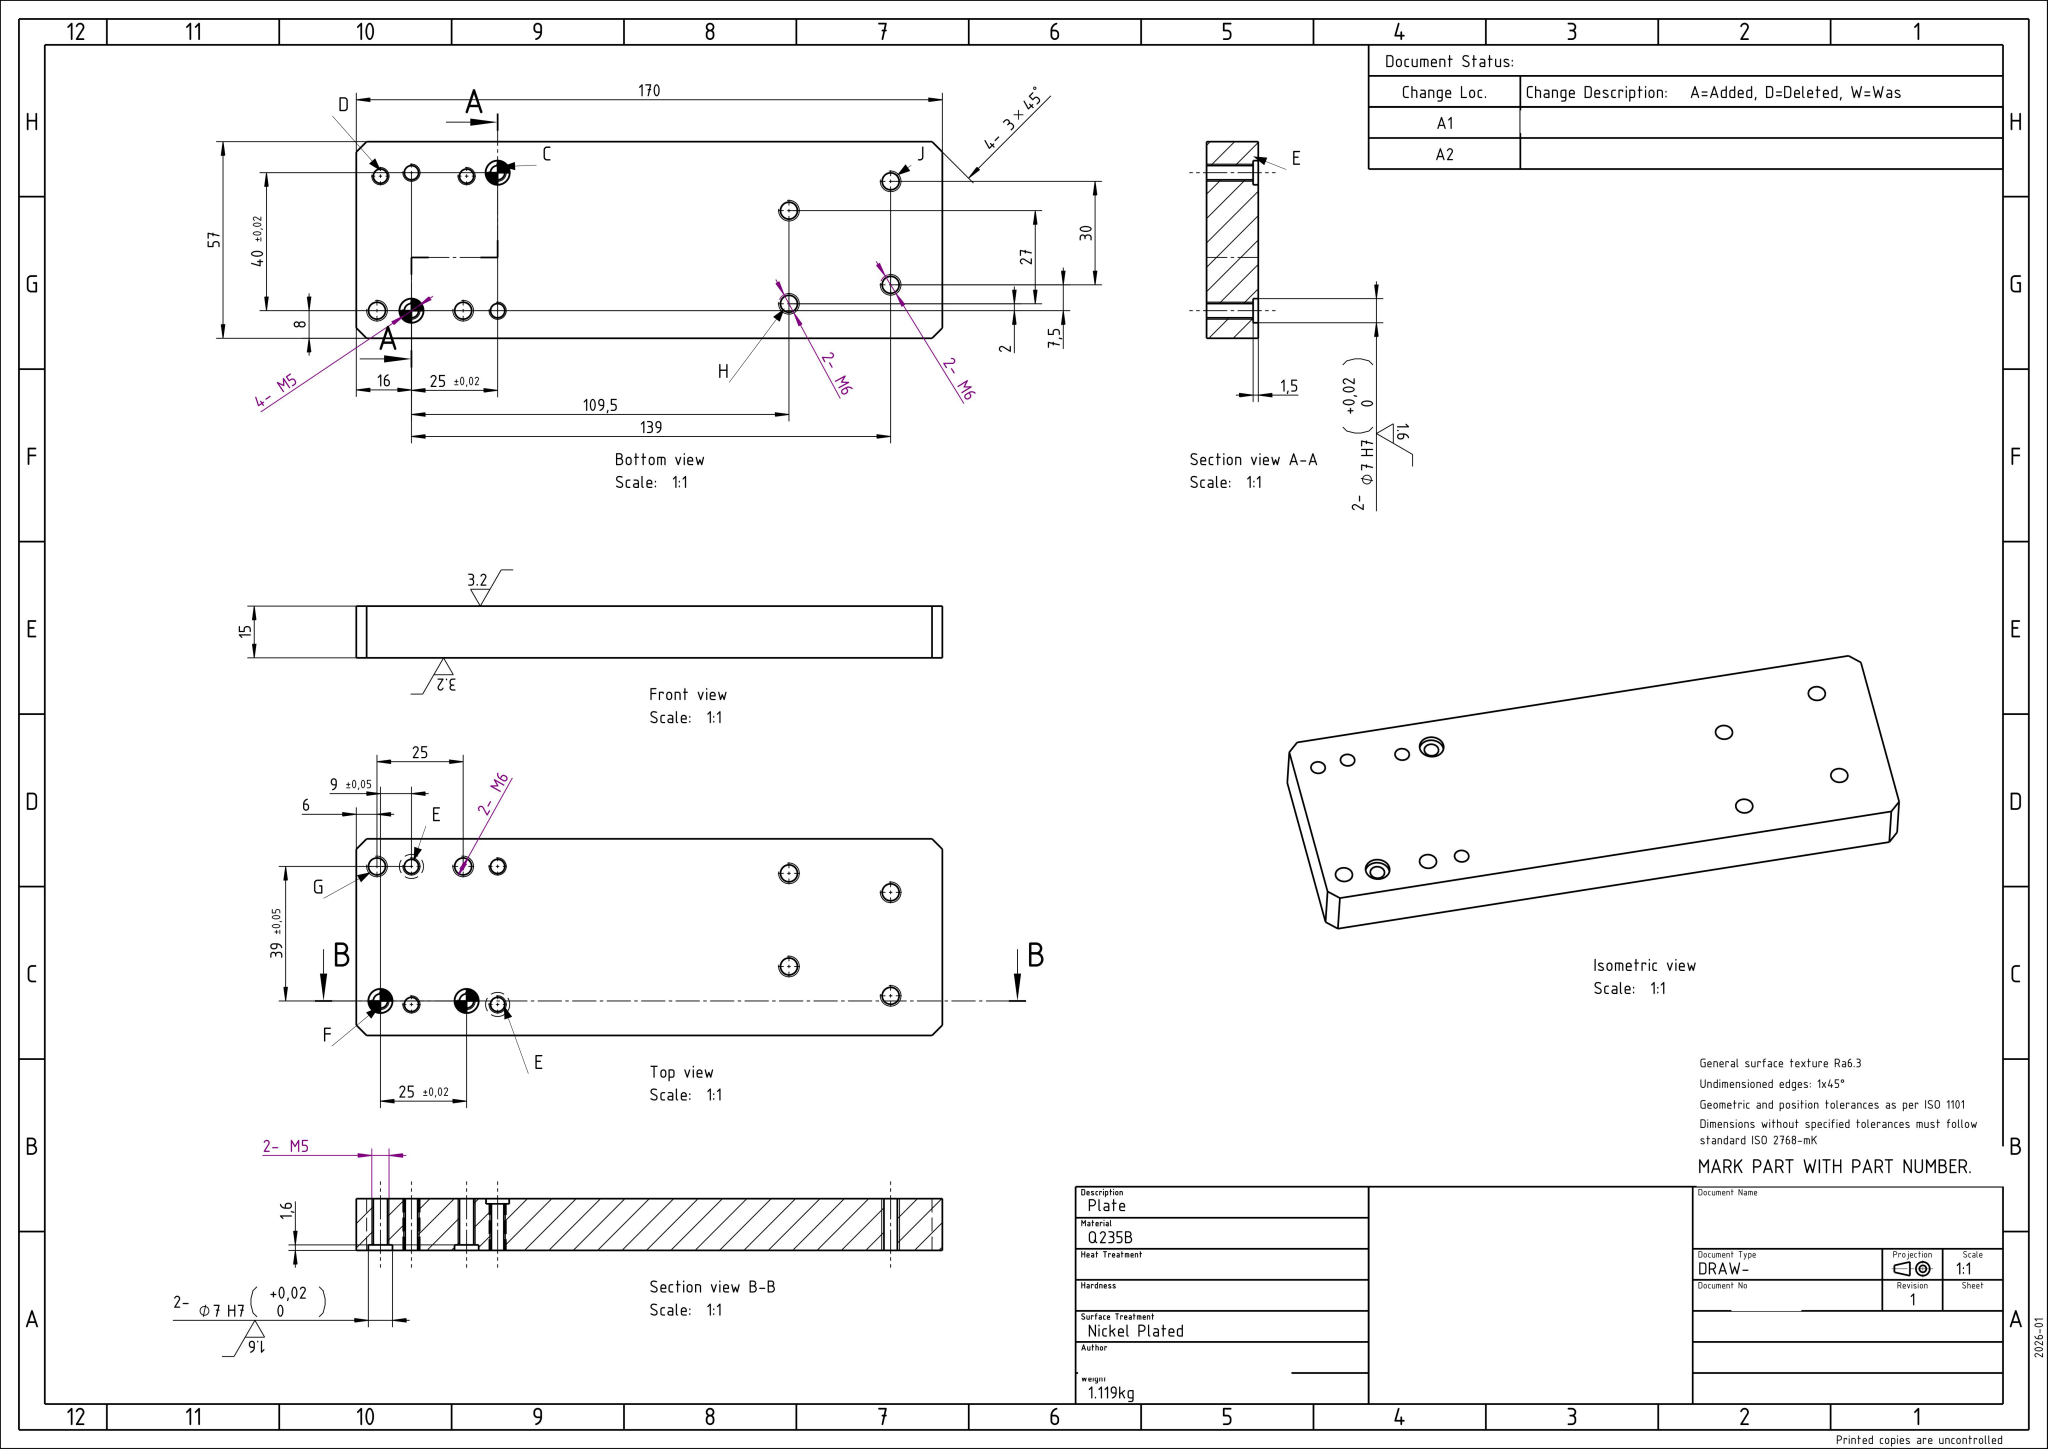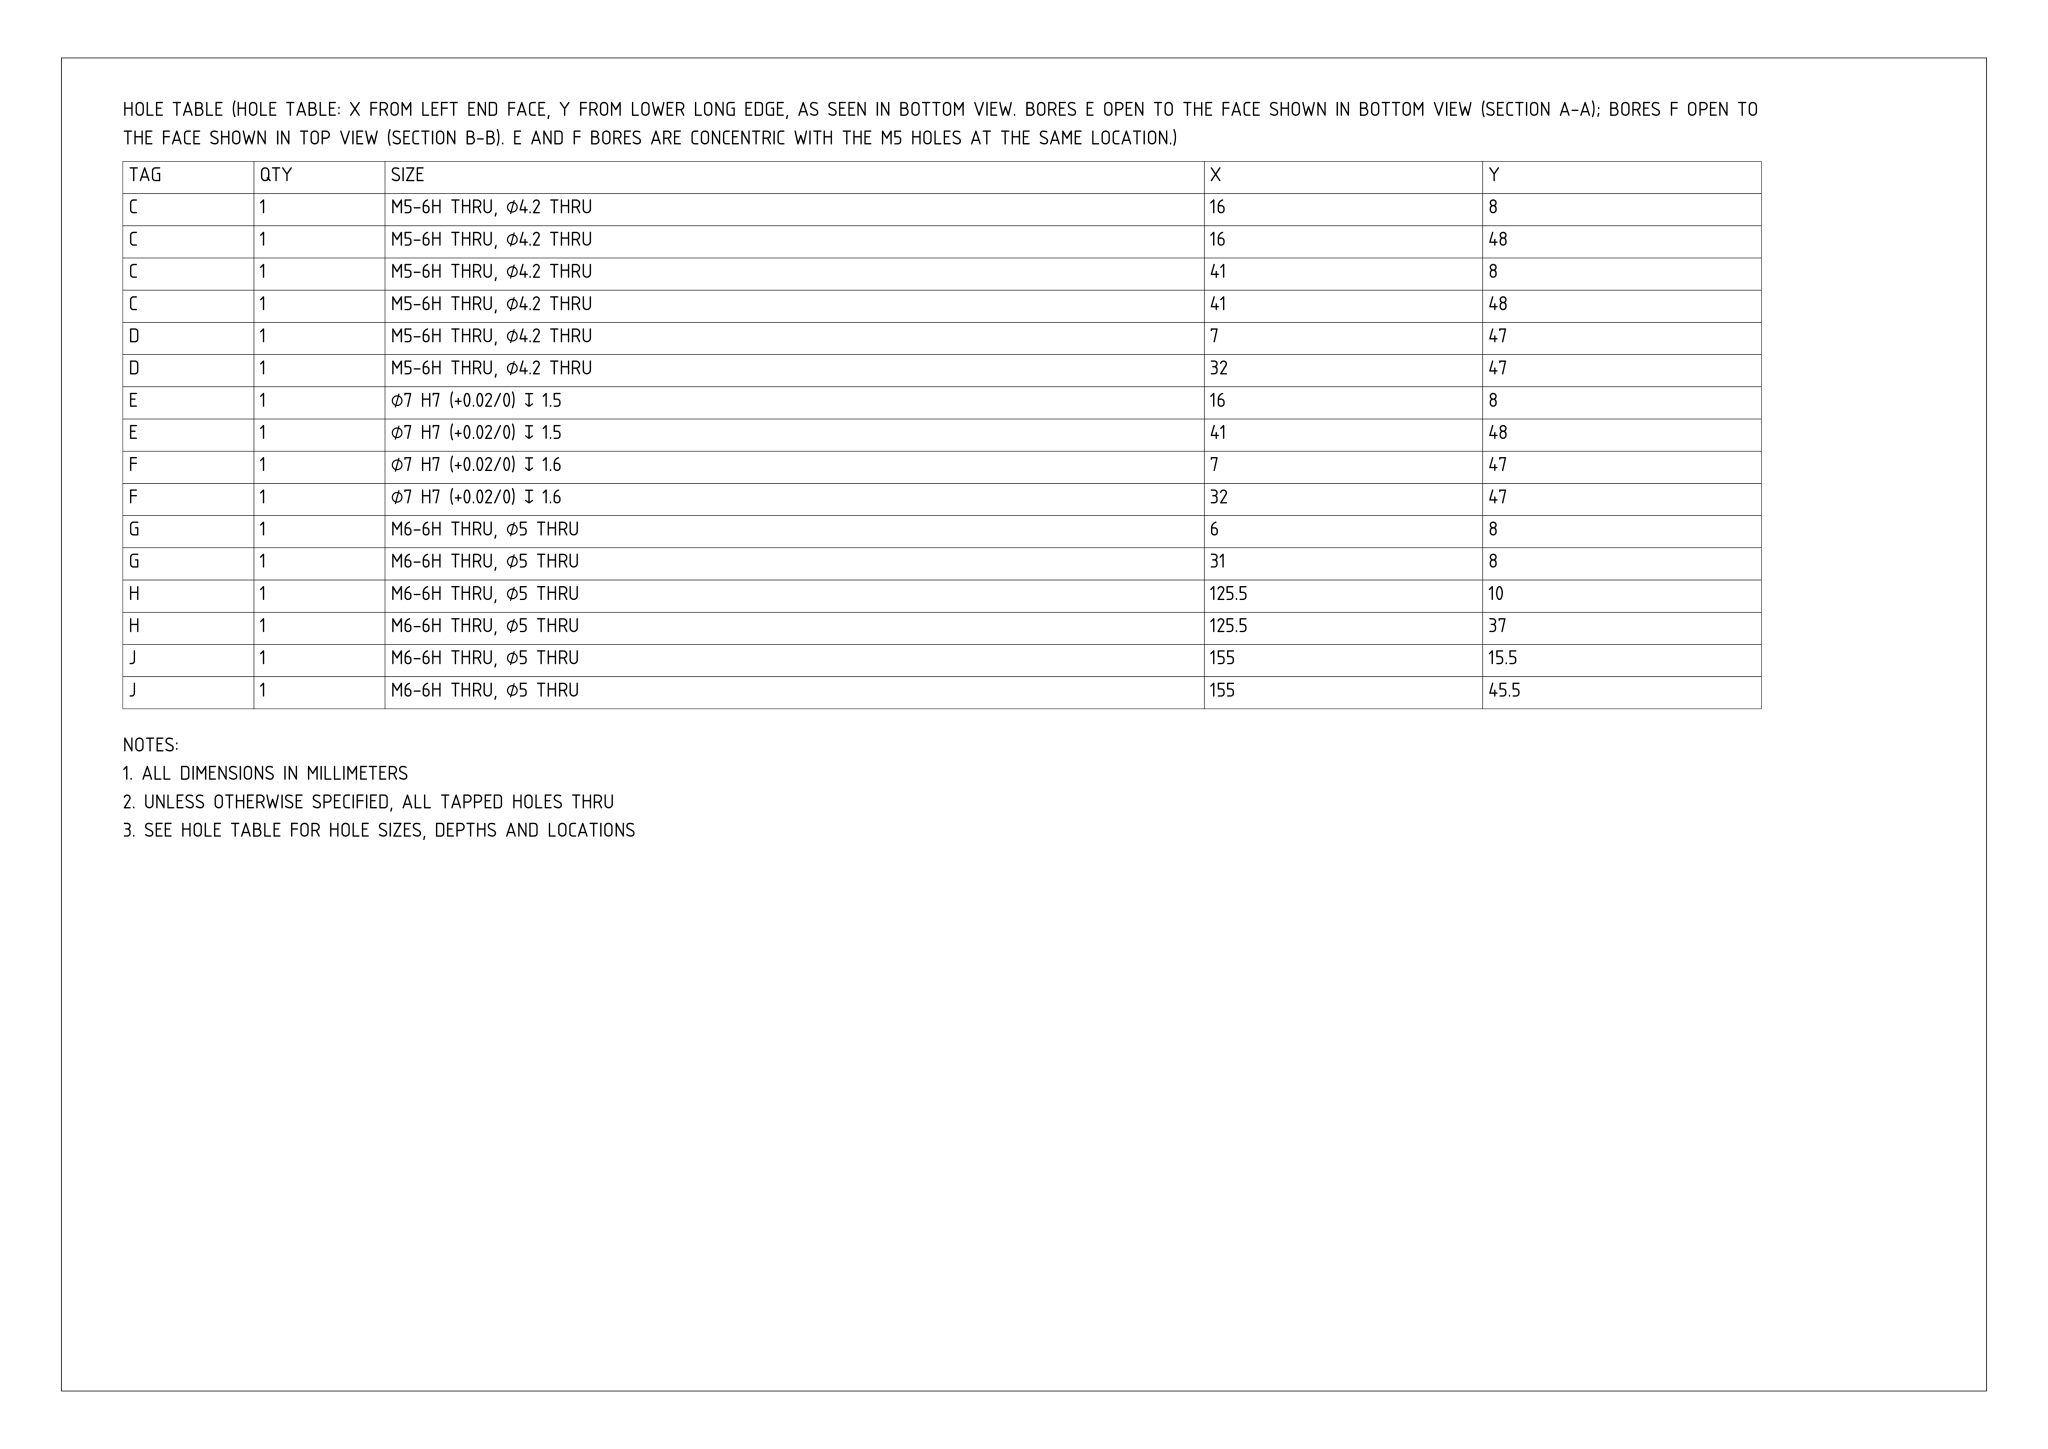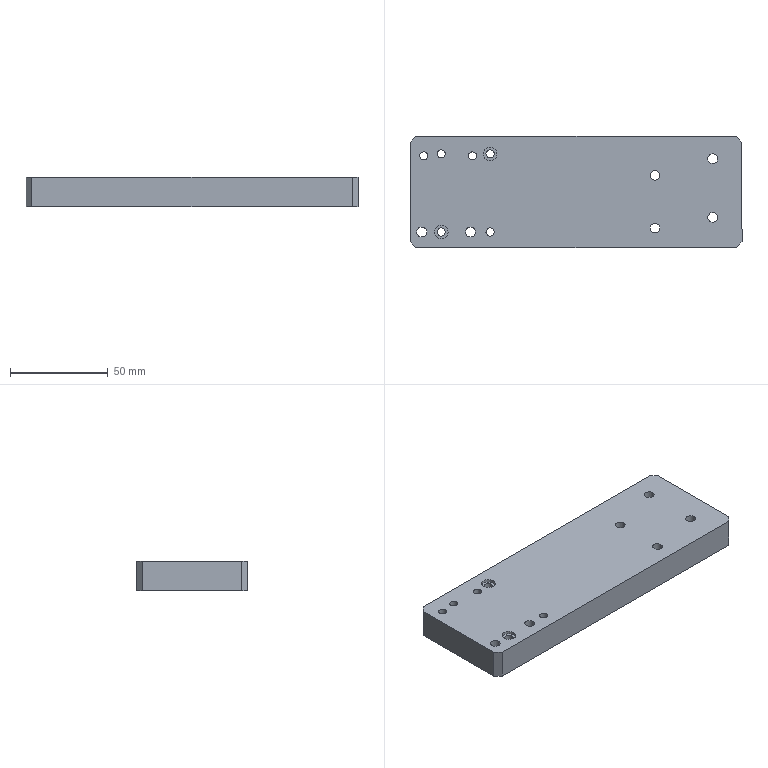Part | NX | mm | 1 solid | 30 faces | box 170 x 57 x 15 mm | volume 141913 mm3 | cylinder 16 | plane 14 | commonest cylinder face diameters 4.2 x6 5 x6 7 x4
STEP:
#1=CARTESIAN_POINT('',(0.,0.,0.));
#2=DIRECTION('',(0.,0.,1.));
#3=DIRECTION('',(1.,0.,0.));
#4=AXIS2_PLACEMENT_3D('',#1,#2,#3);
#5=(LENGTH_UNIT()NAMED_UNIT(*)SI_UNIT(.MILLI.,.METRE.));
#6=UNCERTAINTY_MEASURE_WITH_UNIT(LENGTH_MEASURE(0.00002),#5,'','');
#7=(NAMED_UNIT(*)PLANE_ANGLE_UNIT()SI_UNIT($,.RADIAN.));
#8=PLANE_ANGLE_MEASURE_WITH_UNIT(PLANE_ANGLE_MEASURE(0.01745),#7);
#9=DIMENSIONAL_EXPONENTS(0.,0.,0.,0.,0.,0.,0.);
#10=(CONVERSION_BASED_UNIT('',#8)NAMED_UNIT(#9)PLANE_ANGLE_UNIT());
#11=(NAMED_UNIT(*)SI_UNIT($,.STERADIAN.)SOLID_ANGLE_UNIT());
#12=(GEOMETRIC_REPRESENTATION_CONTEXT(3)GLOBAL_UNCERTAINTY_ASSIGNED_CONTEXT((#6))GLOBAL_UNIT_ASSIGNED_CONTEXT((#5,#10,#11))REPRESENTATION_CONTEXT('',''));
#13=SHAPE_REPRESENTATION('',(#4),#12);
#14=CARTESIAN_POINT('',(-85.,25.5,15.));
#15=VERTEX_POINT('',#14);
#16=CARTESIAN_POINT('',(-85.,-25.5,15.));
#17=VERTEX_POINT('',#16);
#18=CARTESIAN_POINT('',(-85.,28.5,15.));
#19=DIRECTION('',(0.,-1.,0.));
#20=VECTOR('',#19,1.);
#21=LINE('',#18,#20);
#22=EDGE_CURVE('',#15,#17,#21,.T.);
#23=ORIENTED_EDGE('',*,*,#22,.F.);
#24=CARTESIAN_POINT('',(-85.,25.5,0.));
#25=VERTEX_POINT('',#24);
#26=CARTESIAN_POINT('',(-85.,25.5,15.));
#27=DIRECTION('',(0.,0.,-1.));
#28=VECTOR('',#27,1.);
#29=LINE('',#26,#28);
#30=EDGE_CURVE('',#15,#25,#29,.T.);
#31=ORIENTED_EDGE('',*,*,#30,.T.);
#32=CARTESIAN_POINT('',(-85.,-25.5,0.));
#33=VERTEX_POINT('',#32);
#34=CARTESIAN_POINT('',(-85.,28.5,0.));
#35=DIRECTION('',(0.,-1.,0.));
#36=VECTOR('',#35,1.);
#37=LINE('',#34,#36);
#38=EDGE_CURVE('',#25,#33,#37,.T.);
#39=ORIENTED_EDGE('',*,*,#38,.T.);
#40=CARTESIAN_POINT('',(-85.,-25.5,15.));
#41=DIRECTION('',(0.,0.,1.));
#42=VECTOR('',#41,1.);
#43=LINE('',#40,#42);
#44=EDGE_CURVE('',#33,#17,#43,.T.);
#45=ORIENTED_EDGE('',*,*,#44,.T.);
#46=EDGE_LOOP('',(#23,#31,#39,#45));
#47=FACE_OUTER_BOUND('',#46,.T.);
#48=CARTESIAN_POINT('',(-85.,28.5,15.));
#49=DIRECTION('',(1.,0.,0.));
#50=DIRECTION('',(-0.,1.,0.));
#51=AXIS2_PLACEMENT_3D('',#48,#49,#50);
#52=PLANE('',#51);
#53=ADVANCED_FACE('',(#47),#52,.F.);
#54=CARTESIAN_POINT('',(-82.,-28.5,0.));
#55=VERTEX_POINT('',#54);
#56=CARTESIAN_POINT('',(82.,-28.5,0.));
#57=VERTEX_POINT('',#56);
#58=CARTESIAN_POINT('',(-85.,-28.5,0.));
#59=DIRECTION('',(1.,0.,0.));
#60=VECTOR('',#59,1.);
#61=LINE('',#58,#60);
#62=EDGE_CURVE('',#55,#57,#61,.T.);
#63=ORIENTED_EDGE('',*,*,#62,.T.);
#64=CARTESIAN_POINT('',(82.,-28.5,15.));
#65=VERTEX_POINT('',#64);
#66=CARTESIAN_POINT('',(82.,-28.5,15.));
#67=DIRECTION('',(0.,0.,1.));
#68=VECTOR('',#67,1.);
#69=LINE('',#66,#68);
#70=EDGE_CURVE('',#57,#65,#69,.T.);
#71=ORIENTED_EDGE('',*,*,#70,.T.);
#72=CARTESIAN_POINT('',(-82.,-28.5,15.));
#73=VERTEX_POINT('',#72);
#74=CARTESIAN_POINT('',(-85.,-28.5,15.));
#75=DIRECTION('',(1.,0.,0.));
#76=VECTOR('',#75,1.);
#77=LINE('',#74,#76);
#78=EDGE_CURVE('',#73,#65,#77,.T.);
#79=ORIENTED_EDGE('',*,*,#78,.F.);
#80=CARTESIAN_POINT('',(-82.,-28.5,15.));
#81=DIRECTION('',(0.,0.,-1.));
#82=VECTOR('',#81,1.);
#83=LINE('',#80,#82);
#84=EDGE_CURVE('',#73,#55,#83,.T.);
#85=ORIENTED_EDGE('',*,*,#84,.T.);
#86=EDGE_LOOP('',(#63,#71,#79,#85));
#87=FACE_OUTER_BOUND('',#86,.T.);
#88=CARTESIAN_POINT('',(-85.,-28.5,15.));
#89=DIRECTION('',(0.,1.,0.));
#90=DIRECTION('',(0.,0.,1.));
#91=AXIS2_PLACEMENT_3D('',#88,#89,#90);
#92=PLANE('',#91);
#93=ADVANCED_FACE('',(#87),#92,.F.);
#94=CARTESIAN_POINT('',(85.,-25.5,15.));
#95=VERTEX_POINT('',#94);
#96=CARTESIAN_POINT('',(85.,25.5,15.));
#97=VERTEX_POINT('',#96);
#98=CARTESIAN_POINT('',(85.,-28.5,15.));
#99=DIRECTION('',(-0.,1.,0.));
#100=VECTOR('',#99,1.);
#101=LINE('',#98,#100);
#102=EDGE_CURVE('',#95,#97,#101,.T.);
#103=ORIENTED_EDGE('',*,*,#102,.F.);
#104=CARTESIAN_POINT('',(85.,-25.5,0.));
#105=VERTEX_POINT('',#104);
#106=CARTESIAN_POINT('',(85.,-25.5,15.));
#107=DIRECTION('',(0.,0.,-1.));
#108=VECTOR('',#107,1.);
#109=LINE('',#106,#108);
#110=EDGE_CURVE('',#95,#105,#109,.T.);
#111=ORIENTED_EDGE('',*,*,#110,.T.);
#112=CARTESIAN_POINT('',(85.,25.5,0.));
#113=VERTEX_POINT('',#112);
#114=CARTESIAN_POINT('',(85.,-28.5,0.));
#115=DIRECTION('',(-0.,1.,0.));
#116=VECTOR('',#115,1.);
#117=LINE('',#114,#116);
#118=EDGE_CURVE('',#105,#113,#117,.T.);
#119=ORIENTED_EDGE('',*,*,#118,.T.);
#120=CARTESIAN_POINT('',(85.,25.5,15.));
#121=DIRECTION('',(0.,0.,1.));
#122=VECTOR('',#121,1.);
#123=LINE('',#120,#122);
#124=EDGE_CURVE('',#113,#97,#123,.T.);
#125=ORIENTED_EDGE('',*,*,#124,.T.);
#126=EDGE_LOOP('',(#103,#111,#119,#125));
#127=FACE_OUTER_BOUND('',#126,.T.);
#128=CARTESIAN_POINT('',(85.,-28.5,15.));
#129=DIRECTION('',(-1.,-0.,0.));
#130=DIRECTION('',(0.,-1.,0.));
#131=AXIS2_PLACEMENT_3D('',#128,#129,#130);
#132=PLANE('',#131);
#133=ADVANCED_FACE('',(#127),#132,.F.);
#134=CARTESIAN_POINT('',(82.,28.5,0.));
#135=VERTEX_POINT('',#134);
#136=CARTESIAN_POINT('',(-82.,28.5,0.));
#137=VERTEX_POINT('',#136);
#138=CARTESIAN_POINT('',(85.,28.5,0.));
#139=DIRECTION('',(-1.,0.,0.));
#140=VECTOR('',#139,1.);
#141=LINE('',#138,#140);
#142=EDGE_CURVE('',#135,#137,#141,.T.);
#143=ORIENTED_EDGE('',*,*,#142,.T.);
#144=CARTESIAN_POINT('',(-82.,28.5,15.));
#145=VERTEX_POINT('',#144);
#146=CARTESIAN_POINT('',(-82.,28.5,15.));
#147=DIRECTION('',(0.,0.,1.));
#148=VECTOR('',#147,1.);
#149=LINE('',#146,#148);
#150=EDGE_CURVE('',#137,#145,#149,.T.);
#151=ORIENTED_EDGE('',*,*,#150,.T.);
#152=CARTESIAN_POINT('',(82.,28.5,15.));
#153=VERTEX_POINT('',#152);
#154=CARTESIAN_POINT('',(85.,28.5,15.));
#155=DIRECTION('',(-1.,0.,0.));
#156=VECTOR('',#155,1.);
#157=LINE('',#154,#156);
#158=EDGE_CURVE('',#153,#145,#157,.T.);
#159=ORIENTED_EDGE('',*,*,#158,.F.);
#160=CARTESIAN_POINT('',(82.,28.5,15.));
#161=DIRECTION('',(0.,0.,-1.));
#162=VECTOR('',#161,1.);
#163=LINE('',#160,#162);
#164=EDGE_CURVE('',#153,#135,#163,.T.);
#165=ORIENTED_EDGE('',*,*,#164,.T.);
#166=EDGE_LOOP('',(#143,#151,#159,#165));
#167=FACE_OUTER_BOUND('',#166,.T.);
#168=CARTESIAN_POINT('',(85.,28.5,15.));
#169=DIRECTION('',(0.,-1.,0.));
#170=DIRECTION('',(0.,0.,-1.));
#171=AXIS2_PLACEMENT_3D('',#168,#169,#170);
#172=PLANE('',#171);
#173=ADVANCED_FACE('',(#167),#172,.F.);
#174=CARTESIAN_POINT('',(72.5,17.,15.));
#175=VERTEX_POINT('',#174);
#176=CARTESIAN_POINT('',(70.,17.,15.));
#177=DIRECTION('',(0.,0.,1.));
#178=DIRECTION('',(1.,0.,0.));
#179=AXIS2_PLACEMENT_3D('',#176,#177,#178);
#180=CIRCLE('',#179,2.5);
#181=EDGE_CURVE('',#175,#175,#180,.T.);
#182=ORIENTED_EDGE('',*,*,#181,.F.);
#183=EDGE_LOOP('',(#182));
#184=FACE_BOUND('',#183,.T.);
#185=CARTESIAN_POINT('',(72.5,-13.,15.));
#186=VERTEX_POINT('',#185);
#187=CARTESIAN_POINT('',(70.,-13.,15.));
#188=DIRECTION('',(0.,0.,1.));
#189=DIRECTION('',(1.,0.,0.));
#190=AXIS2_PLACEMENT_3D('',#187,#188,#189);
#191=CIRCLE('',#190,2.5);
#192=EDGE_CURVE('',#186,#186,#191,.T.);
#193=ORIENTED_EDGE('',*,*,#192,.F.);
#194=EDGE_LOOP('',(#193));
#195=FACE_BOUND('',#194,.T.);
#196=CARTESIAN_POINT('',(43.,8.5,15.));
#197=VERTEX_POINT('',#196);
#198=CARTESIAN_POINT('',(40.5,8.5,15.));
#199=DIRECTION('',(0.,0.,1.));
#200=DIRECTION('',(1.,0.,0.));
#201=AXIS2_PLACEMENT_3D('',#198,#199,#200);
#202=CIRCLE('',#201,2.5);
#203=EDGE_CURVE('',#197,#197,#202,.T.);
#204=ORIENTED_EDGE('',*,*,#203,.F.);
#205=EDGE_LOOP('',(#204));
#206=FACE_BOUND('',#205,.T.);
#207=CARTESIAN_POINT('',(43.,-18.5,15.));
#208=VERTEX_POINT('',#207);
#209=CARTESIAN_POINT('',(40.5,-18.5,15.));
#210=DIRECTION('',(0.,0.,1.));
#211=DIRECTION('',(1.,0.,0.));
#212=AXIS2_PLACEMENT_3D('',#209,#210,#211);
#213=CIRCLE('',#212,2.5);
#214=EDGE_CURVE('',#208,#208,#213,.T.);
#215=ORIENTED_EDGE('',*,*,#214,.F.);
#216=EDGE_LOOP('',(#215));
#217=FACE_BOUND('',#216,.T.);
#218=CARTESIAN_POINT('',(-50.9,18.5,15.));
#219=VERTEX_POINT('',#218);
#220=CARTESIAN_POINT('',(-53.,18.5,15.));
#221=DIRECTION('',(0.,0.,1.));
#222=DIRECTION('',(1.,0.,0.));
#223=AXIS2_PLACEMENT_3D('',#220,#221,#222);
#224=CIRCLE('',#223,2.1);
#225=EDGE_CURVE('',#219,#219,#224,.T.);
#226=ORIENTED_EDGE('',*,*,#225,.F.);
#227=EDGE_LOOP('',(#226));
#228=FACE_BOUND('',#227,.T.);
#229=CARTESIAN_POINT('',(-75.9,18.5,15.));
#230=VERTEX_POINT('',#229);
#231=CARTESIAN_POINT('',(-78.,18.5,15.));
#232=DIRECTION('',(0.,0.,1.));
#233=DIRECTION('',(1.,0.,0.));
#234=AXIS2_PLACEMENT_3D('',#231,#232,#233);
#235=CIRCLE('',#234,2.1);
#236=EDGE_CURVE('',#230,#230,#235,.T.);
#237=ORIENTED_EDGE('',*,*,#236,.F.);
#238=EDGE_LOOP('',(#237));
#239=FACE_BOUND('',#238,.T.);
#240=CARTESIAN_POINT('',(-56.5,-20.5,15.));
#241=VERTEX_POINT('',#240);
#242=CARTESIAN_POINT('',(-54.,-20.5,15.));
#243=DIRECTION('',(0.,0.,-1.));
#244=DIRECTION('',(-1.,0.,0.));
#245=AXIS2_PLACEMENT_3D('',#242,#243,#244);
#246=CIRCLE('',#245,2.5);
#247=EDGE_CURVE('',#241,#241,#246,.T.);
#248=ORIENTED_EDGE('',*,*,#247,.T.);
#249=EDGE_LOOP('',(#248));
#250=FACE_BOUND('',#249,.T.);
#251=CARTESIAN_POINT('',(-81.5,-20.5,15.));
#252=VERTEX_POINT('',#251);
#253=CARTESIAN_POINT('',(-79.,-20.5,15.));
#254=DIRECTION('',(0.,0.,-1.));
#255=DIRECTION('',(-1.,0.,0.));
#256=AXIS2_PLACEMENT_3D('',#253,#254,#255);
#257=CIRCLE('',#256,2.5);
#258=EDGE_CURVE('',#252,#252,#257,.T.);
#259=ORIENTED_EDGE('',*,*,#258,.T.);
#260=EDGE_LOOP('',(#259));
#261=FACE_BOUND('',#260,.T.);
#262=CARTESIAN_POINT('',(-46.1,-20.5,15.));
#263=VERTEX_POINT('',#262);
#264=CARTESIAN_POINT('',(-44.,-20.5,15.));
#265=DIRECTION('',(0.,0.,-1.));
#266=DIRECTION('',(-1.,0.,0.));
#267=AXIS2_PLACEMENT_3D('',#264,#265,#266);
#268=CIRCLE('',#267,2.1);
#269=EDGE_CURVE('',#263,#263,#268,.T.);
#270=ORIENTED_EDGE('',*,*,#269,.T.);
#271=EDGE_LOOP('',(#270));
#272=FACE_BOUND('',#271,.T.);
#273=CARTESIAN_POINT('',(-71.1,19.5,15.));
#274=VERTEX_POINT('',#273);
#275=CARTESIAN_POINT('',(-69.,19.5,15.));
#276=DIRECTION('',(0.,0.,-1.));
#277=DIRECTION('',(-1.,0.,0.));
#278=AXIS2_PLACEMENT_3D('',#275,#276,#277);
#279=CIRCLE('',#278,2.1);
#280=EDGE_CURVE('',#274,#274,#279,.T.);
#281=ORIENTED_EDGE('',*,*,#280,.T.);
#282=EDGE_LOOP('',(#281));
#283=FACE_BOUND('',#282,.T.);
#284=CARTESIAN_POINT('',(-47.5,19.5,15.));
#285=VERTEX_POINT('',#284);
#286=CARTESIAN_POINT('',(-44.,19.5,15.));
#287=DIRECTION('',(0.,0.,-1.));
#288=DIRECTION('',(-1.,0.,0.));
#289=AXIS2_PLACEMENT_3D('',#286,#287,#288);
#290=CIRCLE('',#289,3.5);
#291=EDGE_CURVE('',#285,#285,#290,.T.);
#292=ORIENTED_EDGE('',*,*,#291,.T.);
#293=EDGE_LOOP('',(#292));
#294=FACE_BOUND('',#293,.T.);
#295=CARTESIAN_POINT('',(-72.5,-20.5,15.));
#296=VERTEX_POINT('',#295);
#297=CARTESIAN_POINT('',(-69.,-20.5,15.));
#298=DIRECTION('',(0.,0.,-1.));
#299=DIRECTION('',(-1.,0.,0.));
#300=AXIS2_PLACEMENT_3D('',#297,#298,#299);
#301=CIRCLE('',#300,3.5);
#302=EDGE_CURVE('',#296,#296,#301,.T.);
#303=ORIENTED_EDGE('',*,*,#302,.T.);
#304=EDGE_LOOP('',(#303));
#305=FACE_BOUND('',#304,.T.);
#306=ORIENTED_EDGE('',*,*,#158,.T.);
#307=CARTESIAN_POINT('',(-55.25,55.25,15.));
#308=DIRECTION('',(-0.7071,-0.7071,0.));
#309=VECTOR('',#308,1.);
#310=LINE('',#307,#309);
#311=EDGE_CURVE('',#145,#15,#310,.T.);
#312=ORIENTED_EDGE('',*,*,#311,.T.);
#313=ORIENTED_EDGE('',*,*,#22,.T.);
#314=CARTESIAN_POINT('',(-55.25,-55.25,15.));
#315=DIRECTION('',(0.7071,-0.7071,0.));
#316=VECTOR('',#315,1.);
#317=LINE('',#314,#316);
#318=EDGE_CURVE('',#17,#73,#317,.T.);
#319=ORIENTED_EDGE('',*,*,#318,.T.);
#320=ORIENTED_EDGE('',*,*,#78,.T.);
#321=CARTESIAN_POINT('',(55.25,-55.25,15.));
#322=DIRECTION('',(0.7071,0.7071,0.));
#323=VECTOR('',#322,1.);
#324=LINE('',#321,#323);
#325=EDGE_CURVE('',#65,#95,#324,.T.);
#326=ORIENTED_EDGE('',*,*,#325,.T.);
#327=ORIENTED_EDGE('',*,*,#102,.T.);
#328=CARTESIAN_POINT('',(55.25,55.25,15.));
#329=DIRECTION('',(-0.7071,0.7071,0.));
#330=VECTOR('',#329,1.);
#331=LINE('',#328,#330);
#332=EDGE_CURVE('',#97,#153,#331,.T.);
#333=ORIENTED_EDGE('',*,*,#332,.T.);
#334=EDGE_LOOP('',(#306,#312,#313,#319,#320,#326,#327,#333));
#335=FACE_BOUND('',#334,.T.);
#336=CARTESIAN_POINT('',(0.,0.,15.));
#337=DIRECTION('',(0.,0.,1.));
#338=DIRECTION('',(1.,0.,0.));
#339=AXIS2_PLACEMENT_3D('',#336,#337,#338);
#340=PLANE('',#339);
#341=ADVANCED_FACE('',(#184,#195,#206,#217,#228,#239,#250,#261,#272,#283,#294,#305,#335),#340,.T.);
#342=CARTESIAN_POINT('',(72.5,17.,0.));
#343=VERTEX_POINT('',#342);
#344=CARTESIAN_POINT('',(70.,17.,0.));
#345=DIRECTION('',(0.,0.,1.));
#346=DIRECTION('',(1.,0.,0.));
#347=AXIS2_PLACEMENT_3D('',#344,#345,#346);
#348=CIRCLE('',#347,2.5);
#349=EDGE_CURVE('',#343,#343,#348,.T.);
#350=ORIENTED_EDGE('',*,*,#349,.T.);
#351=EDGE_LOOP('',(#350));
#352=FACE_BOUND('',#351,.T.);
#353=CARTESIAN_POINT('',(72.5,-13.,0.));
#354=VERTEX_POINT('',#353);
#355=CARTESIAN_POINT('',(70.,-13.,0.));
#356=DIRECTION('',(0.,0.,1.));
#357=DIRECTION('',(1.,0.,0.));
#358=AXIS2_PLACEMENT_3D('',#355,#356,#357);
#359=CIRCLE('',#358,2.5);
#360=EDGE_CURVE('',#354,#354,#359,.T.);
#361=ORIENTED_EDGE('',*,*,#360,.T.);
#362=EDGE_LOOP('',(#361));
#363=FACE_BOUND('',#362,.T.);
#364=CARTESIAN_POINT('',(43.,8.5,0.));
#365=VERTEX_POINT('',#364);
#366=CARTESIAN_POINT('',(40.5,8.5,0.));
#367=DIRECTION('',(0.,0.,1.));
#368=DIRECTION('',(1.,0.,0.));
#369=AXIS2_PLACEMENT_3D('',#366,#367,#368);
#370=CIRCLE('',#369,2.5);
#371=EDGE_CURVE('',#365,#365,#370,.T.);
#372=ORIENTED_EDGE('',*,*,#371,.T.);
#373=EDGE_LOOP('',(#372));
#374=FACE_BOUND('',#373,.T.);
#375=CARTESIAN_POINT('',(43.,-18.5,0.));
#376=VERTEX_POINT('',#375);
#377=CARTESIAN_POINT('',(40.5,-18.5,0.));
#378=DIRECTION('',(0.,0.,1.));
#379=DIRECTION('',(1.,0.,0.));
#380=AXIS2_PLACEMENT_3D('',#377,#378,#379);
#381=CIRCLE('',#380,2.5);
#382=EDGE_CURVE('',#376,#376,#381,.T.);
#383=ORIENTED_EDGE('',*,*,#382,.T.);
#384=EDGE_LOOP('',(#383));
#385=FACE_BOUND('',#384,.T.);
#386=CARTESIAN_POINT('',(-51.5,-20.5,0.));
#387=VERTEX_POINT('',#386);
#388=CARTESIAN_POINT('',(-54.,-20.5,0.));
#389=DIRECTION('',(0.,0.,1.));
#390=DIRECTION('',(1.,0.,0.));
#391=AXIS2_PLACEMENT_3D('',#388,#389,#390);
#392=CIRCLE('',#391,2.5);
#393=EDGE_CURVE('',#387,#387,#392,.T.);
#394=ORIENTED_EDGE('',*,*,#393,.T.);
#395=EDGE_LOOP('',(#394));
#396=FACE_BOUND('',#395,.T.);
#397=CARTESIAN_POINT('',(-76.5,-20.5,0.));
#398=VERTEX_POINT('',#397);
#399=CARTESIAN_POINT('',(-79.,-20.5,0.));
#400=DIRECTION('',(0.,0.,1.));
#401=DIRECTION('',(1.,0.,0.));
#402=AXIS2_PLACEMENT_3D('',#399,#400,#401);
#403=CIRCLE('',#402,2.5);
#404=EDGE_CURVE('',#398,#398,#403,.T.);
#405=ORIENTED_EDGE('',*,*,#404,.T.);
#406=EDGE_LOOP('',(#405));
#407=FACE_BOUND('',#406,.T.);
#408=CARTESIAN_POINT('',(-49.5,18.5,0.));
#409=VERTEX_POINT('',#408);
#410=CARTESIAN_POINT('',(-53.,18.5,0.));
#411=DIRECTION('',(0.,0.,1.));
#412=DIRECTION('',(1.,0.,0.));
#413=AXIS2_PLACEMENT_3D('',#410,#411,#412);
#414=CIRCLE('',#413,3.5);
#415=EDGE_CURVE('',#409,#409,#414,.T.);
#416=ORIENTED_EDGE('',*,*,#415,.T.);
#417=EDGE_LOOP('',(#416));
#418=FACE_BOUND('',#417,.T.);
#419=CARTESIAN_POINT('',(-74.5,18.5,0.));
#420=VERTEX_POINT('',#419);
#421=CARTESIAN_POINT('',(-78.,18.5,0.));
#422=DIRECTION('',(0.,0.,1.));
#423=DIRECTION('',(1.,0.,0.));
#424=AXIS2_PLACEMENT_3D('',#421,#422,#423);
#425=CIRCLE('',#424,3.5);
#426=EDGE_CURVE('',#420,#420,#425,.T.);
#427=ORIENTED_EDGE('',*,*,#426,.T.);
#428=EDGE_LOOP('',(#427));
#429=FACE_BOUND('',#428,.T.);
#430=CARTESIAN_POINT('',(-41.9,19.5,0.));
#431=VERTEX_POINT('',#430);
#432=CARTESIAN_POINT('',(-44.,19.5,0.));
#433=DIRECTION('',(0.,0.,1.));
#434=DIRECTION('',(1.,0.,0.));
#435=AXIS2_PLACEMENT_3D('',#432,#433,#434);
#436=CIRCLE('',#435,2.1);
#437=EDGE_CURVE('',#431,#431,#436,.T.);
#438=ORIENTED_EDGE('',*,*,#437,.T.);
#439=EDGE_LOOP('',(#438));
#440=FACE_BOUND('',#439,.T.);
#441=CARTESIAN_POINT('',(-66.9,-20.5,0.));
#442=VERTEX_POINT('',#441);
#443=CARTESIAN_POINT('',(-69.,-20.5,0.));
#444=DIRECTION('',(0.,0.,1.));
#445=DIRECTION('',(1.,0.,0.));
#446=AXIS2_PLACEMENT_3D('',#443,#444,#445);
#447=CIRCLE('',#446,2.1);
#448=EDGE_CURVE('',#442,#442,#447,.T.);
#449=ORIENTED_EDGE('',*,*,#448,.T.);
#450=EDGE_LOOP('',(#449));
#451=FACE_BOUND('',#450,.T.);
#452=CARTESIAN_POINT('',(-41.9,-20.5,0.));
#453=VERTEX_POINT('',#452);
#454=CARTESIAN_POINT('',(-44.,-20.5,0.));
#455=DIRECTION('',(0.,0.,1.));
#456=DIRECTION('',(1.,0.,0.));
#457=AXIS2_PLACEMENT_3D('',#454,#455,#456);
#458=CIRCLE('',#457,2.1);
#459=EDGE_CURVE('',#453,#453,#458,.T.);
#460=ORIENTED_EDGE('',*,*,#459,.T.);
#461=EDGE_LOOP('',(#460));
#462=FACE_BOUND('',#461,.T.);
#463=CARTESIAN_POINT('',(-66.9,19.5,0.));
#464=VERTEX_POINT('',#463);
#465=CARTESIAN_POINT('',(-69.,19.5,0.));
#466=DIRECTION('',(0.,0.,1.));
#467=DIRECTION('',(1.,0.,0.));
#468=AXIS2_PLACEMENT_3D('',#465,#466,#467);
#469=CIRCLE('',#468,2.1);
#470=EDGE_CURVE('',#464,#464,#469,.T.);
#471=ORIENTED_EDGE('',*,*,#470,.T.);
#472=EDGE_LOOP('',(#471));
#473=FACE_BOUND('',#472,.T.);
#474=ORIENTED_EDGE('',*,*,#38,.F.);
#475=CARTESIAN_POINT('',(-85.,25.5,0.));
#476=DIRECTION('',(0.7071,0.7071,0.));
#477=VECTOR('',#476,1.);
#478=LINE('',#475,#477);
#479=EDGE_CURVE('',#25,#137,#478,.T.);
#480=ORIENTED_EDGE('',*,*,#479,.T.);
#481=ORIENTED_EDGE('',*,*,#142,.F.);
#482=CARTESIAN_POINT('',(82.,28.5,0.));
#483=DIRECTION('',(0.7071,-0.7071,0.));
#484=VECTOR('',#483,1.);
#485=LINE('',#482,#484);
#486=EDGE_CURVE('',#135,#113,#485,.T.);
#487=ORIENTED_EDGE('',*,*,#486,.T.);
#488=ORIENTED_EDGE('',*,*,#118,.F.);
#489=CARTESIAN_POINT('',(85.,-25.5,0.));
#490=DIRECTION('',(-0.7071,-0.7071,0.));
#491=VECTOR('',#490,1.);
#492=LINE('',#489,#491);
#493=EDGE_CURVE('',#105,#57,#492,.T.);
#494=ORIENTED_EDGE('',*,*,#493,.T.);
#495=ORIENTED_EDGE('',*,*,#62,.F.);
#496=CARTESIAN_POINT('',(-82.,-28.5,0.));
#497=DIRECTION('',(-0.7071,0.7071,0.));
#498=VECTOR('',#497,1.);
#499=LINE('',#496,#498);
#500=EDGE_CURVE('',#55,#33,#499,.T.);
#501=ORIENTED_EDGE('',*,*,#500,.T.);
#502=EDGE_LOOP('',(#474,#480,#481,#487,#488,#494,#495,#501));
#503=FACE_BOUND('',#502,.T.);
#504=CARTESIAN_POINT('',(0.,0.,0.));
#505=DIRECTION('',(0.,0.,1.));
#506=DIRECTION('',(1.,0.,0.));
#507=AXIS2_PLACEMENT_3D('',#504,#505,#506);
#508=PLANE('',#507);
#509=ADVANCED_FACE('',(#352,#363,#374,#385,#396,#407,#418,#429,#440,#451,#462,#473,#503),#508,.F.);
#510=ORIENTED_EDGE('',*,*,#311,.F.);
#511=ORIENTED_EDGE('',*,*,#150,.F.);
#512=ORIENTED_EDGE('',*,*,#479,.F.);
#513=ORIENTED_EDGE('',*,*,#30,.F.);
#514=EDGE_LOOP('',(#510,#511,#512,#513));
#515=FACE_OUTER_BOUND('',#514,.T.);
#516=CARTESIAN_POINT('',(-85.,25.5,15.));
#517=DIRECTION('',(0.7071,-0.7071,0.));
#518=DIRECTION('',(0.,0.,-1.));
#519=AXIS2_PLACEMENT_3D('',#516,#517,#518);
#520=PLANE('',#519);
#521=ADVANCED_FACE('',(#515),#520,.F.);
#522=ORIENTED_EDGE('',*,*,#325,.F.);
#523=ORIENTED_EDGE('',*,*,#70,.F.);
#524=ORIENTED_EDGE('',*,*,#493,.F.);
#525=ORIENTED_EDGE('',*,*,#110,.F.);
#526=EDGE_LOOP('',(#522,#523,#524,#525));
#527=FACE_OUTER_BOUND('',#526,.T.);
#528=CARTESIAN_POINT('',(85.,-25.5,15.));
#529=DIRECTION('',(-0.7071,0.7071,0.));
#530=DIRECTION('',(0.,0.,-1.));
#531=AXIS2_PLACEMENT_3D('',#528,#529,#530);
#532=PLANE('',#531);
#533=ADVANCED_FACE('',(#527),#532,.F.);
#534=ORIENTED_EDGE('',*,*,#332,.F.);
#535=ORIENTED_EDGE('',*,*,#124,.F.);
#536=ORIENTED_EDGE('',*,*,#486,.F.);
#537=ORIENTED_EDGE('',*,*,#164,.F.);
#538=EDGE_LOOP('',(#534,#535,#536,#537));
#539=FACE_OUTER_BOUND('',#538,.T.);
#540=CARTESIAN_POINT('',(82.,28.5,15.));
#541=DIRECTION('',(-0.7071,-0.7071,0.));
#542=DIRECTION('',(0.,0.,-1.));
#543=AXIS2_PLACEMENT_3D('',#540,#541,#542);
#544=PLANE('',#543);
#545=ADVANCED_FACE('',(#539),#544,.F.);
#546=ORIENTED_EDGE('',*,*,#318,.F.);
#547=ORIENTED_EDGE('',*,*,#44,.F.);
#548=ORIENTED_EDGE('',*,*,#500,.F.);
#549=ORIENTED_EDGE('',*,*,#84,.F.);
#550=EDGE_LOOP('',(#546,#547,#548,#549));
#551=FACE_OUTER_BOUND('',#550,.T.);
#552=CARTESIAN_POINT('',(-82.,-28.5,15.));
#553=DIRECTION('',(0.7071,0.7071,0.));
#554=DIRECTION('',(0.,0.,-1.));
#555=AXIS2_PLACEMENT_3D('',#552,#553,#554);
#556=PLANE('',#555);
#557=ADVANCED_FACE('',(#551),#556,.F.);
#558=CARTESIAN_POINT('',(-71.1,-20.5,13.5));
#559=VERTEX_POINT('',#558);
#560=CARTESIAN_POINT('',(-69.,-20.5,13.5));
#561=DIRECTION('',(0.,0.,-1.));
#562=DIRECTION('',(-1.,0.,0.));
#563=AXIS2_PLACEMENT_3D('',#560,#561,#562);
#564=CIRCLE('',#563,2.1);
#565=EDGE_CURVE('',#559,#559,#564,.T.);
#566=ORIENTED_EDGE('',*,*,#565,.T.);
#567=EDGE_LOOP('',(#566));
#568=FACE_BOUND('',#567,.T.);
#569=CARTESIAN_POINT('',(-72.5,-20.5,13.5));
#570=VERTEX_POINT('',#569);
#571=CARTESIAN_POINT('',(-69.,-20.5,13.5));
#572=DIRECTION('',(0.,0.,1.));
#573=DIRECTION('',(-1.,0.,0.));
#574=AXIS2_PLACEMENT_3D('',#571,#572,#573);
#575=CIRCLE('',#574,3.5);
#576=EDGE_CURVE('',#570,#570,#575,.T.);
#577=ORIENTED_EDGE('',*,*,#576,.T.);
#578=EDGE_LOOP('',(#577));
#579=FACE_BOUND('',#578,.T.);
#580=CARTESIAN_POINT('',(-69.,-20.5,13.5));
#581=DIRECTION('',(0.,0.,-1.));
#582=DIRECTION('',(-1.,0.,0.));
#583=AXIS2_PLACEMENT_3D('',#580,#581,#582);
#584=PLANE('',#583);
#585=ADVANCED_FACE('',(#568,#579),#584,.F.);
#586=ORIENTED_EDGE('',*,*,#576,.F.);
#587=EDGE_LOOP('',(#586));
#588=FACE_BOUND('',#587,.T.);
#589=ORIENTED_EDGE('',*,*,#302,.F.);
#590=EDGE_LOOP('',(#589));
#591=FACE_BOUND('',#590,.T.);
#592=CARTESIAN_POINT('',(-69.,-20.5,15.));
#593=DIRECTION('',(0.,0.,-1.));
#594=DIRECTION('',(-1.,0.,0.));
#595=AXIS2_PLACEMENT_3D('',#592,#593,#594);
#596=CYLINDRICAL_SURFACE('',#595,3.5);
#597=ADVANCED_FACE('',(#588,#591),#596,.F.);
#598=CARTESIAN_POINT('',(-46.1,19.5,13.5));
#599=VERTEX_POINT('',#598);
#600=CARTESIAN_POINT('',(-44.,19.5,13.5));
#601=DIRECTION('',(0.,0.,-1.));
#602=DIRECTION('',(-1.,0.,0.));
#603=AXIS2_PLACEMENT_3D('',#600,#601,#602);
#604=CIRCLE('',#603,2.1);
#605=EDGE_CURVE('',#599,#599,#604,.T.);
#606=ORIENTED_EDGE('',*,*,#605,.T.);
#607=EDGE_LOOP('',(#606));
#608=FACE_BOUND('',#607,.T.);
#609=CARTESIAN_POINT('',(-47.5,19.5,13.5));
#610=VERTEX_POINT('',#609);
#611=CARTESIAN_POINT('',(-44.,19.5,13.5));
#612=DIRECTION('',(0.,0.,1.));
#613=DIRECTION('',(-1.,0.,0.));
#614=AXIS2_PLACEMENT_3D('',#611,#612,#613);
#615=CIRCLE('',#614,3.5);
#616=EDGE_CURVE('',#610,#610,#615,.T.);
#617=ORIENTED_EDGE('',*,*,#616,.T.);
#618=EDGE_LOOP('',(#617));
#619=FACE_BOUND('',#618,.T.);
#620=CARTESIAN_POINT('',(-44.,19.5,13.5));
#621=DIRECTION('',(0.,0.,-1.));
#622=DIRECTION('',(-1.,0.,0.));
#623=AXIS2_PLACEMENT_3D('',#620,#621,#622);
#624=PLANE('',#623);
#625=ADVANCED_FACE('',(#608,#619),#624,.F.);
#626=ORIENTED_EDGE('',*,*,#616,.F.);
#627=EDGE_LOOP('',(#626));
#628=FACE_BOUND('',#627,.T.);
#629=ORIENTED_EDGE('',*,*,#291,.F.);
#630=EDGE_LOOP('',(#629));
#631=FACE_BOUND('',#630,.T.);
#632=CARTESIAN_POINT('',(-44.,19.5,15.));
#633=DIRECTION('',(0.,0.,-1.));
#634=DIRECTION('',(-1.,0.,0.));
#635=AXIS2_PLACEMENT_3D('',#632,#633,#634);
#636=CYLINDRICAL_SURFACE('',#635,3.5);
#637=ADVANCED_FACE('',(#628,#631),#636,.F.);
#638=ORIENTED_EDGE('',*,*,#280,.F.);
#639=EDGE_LOOP('',(#638));
#640=FACE_BOUND('',#639,.T.);
#641=ORIENTED_EDGE('',*,*,#470,.F.);
#642=EDGE_LOOP('',(#641));
#643=FACE_BOUND('',#642,.T.);
#644=CARTESIAN_POINT('',(-69.,19.5,15.));
#645=DIRECTION('',(0.,0.,-1.));
#646=DIRECTION('',(-1.,0.,0.));
#647=AXIS2_PLACEMENT_3D('',#644,#645,#646);
#648=CYLINDRICAL_SURFACE('',#647,2.1);
#649=ADVANCED_FACE('',(#640,#643),#648,.F.);
#650=ORIENTED_EDGE('',*,*,#269,.F.);
#651=EDGE_LOOP('',(#650));
#652=FACE_BOUND('',#651,.T.);
#653=ORIENTED_EDGE('',*,*,#459,.F.);
#654=EDGE_LOOP('',(#653));
#655=FACE_BOUND('',#654,.T.);
#656=CARTESIAN_POINT('',(-44.,-20.5,15.));
#657=DIRECTION('',(0.,0.,-1.));
#658=DIRECTION('',(-1.,0.,0.));
#659=AXIS2_PLACEMENT_3D('',#656,#657,#658);
#660=CYLINDRICAL_SURFACE('',#659,2.1);
#661=ADVANCED_FACE('',(#652,#655),#660,.F.);
#662=ORIENTED_EDGE('',*,*,#565,.F.);
#663=EDGE_LOOP('',(#662));
#664=FACE_BOUND('',#663,.T.);
#665=ORIENTED_EDGE('',*,*,#448,.F.);
#666=EDGE_LOOP('',(#665));
#667=FACE_BOUND('',#666,.T.);
#668=CARTESIAN_POINT('',(-69.,-20.5,13.5));
#669=DIRECTION('',(0.,0.,-1.));
#670=DIRECTION('',(-1.,0.,0.));
#671=AXIS2_PLACEMENT_3D('',#668,#669,#670);
#672=CYLINDRICAL_SURFACE('',#671,2.1);
#673=ADVANCED_FACE('',(#664,#667),#672,.F.);
#674=ORIENTED_EDGE('',*,*,#605,.F.);
#675=EDGE_LOOP('',(#674));
#676=FACE_BOUND('',#675,.T.);
#677=ORIENTED_EDGE('',*,*,#437,.F.);
#678=EDGE_LOOP('',(#677));
#679=FACE_BOUND('',#678,.T.);
#680=CARTESIAN_POINT('',(-44.,19.5,13.5));
#681=DIRECTION('',(0.,0.,-1.));
#682=DIRECTION('',(-1.,0.,0.));
#683=AXIS2_PLACEMENT_3D('',#680,#681,#682);
#684=CYLINDRICAL_SURFACE('',#683,2.1);
#685=ADVANCED_FACE('',(#676,#679),#684,.F.);
#686=CARTESIAN_POINT('',(-75.9,18.5,1.6));
#687=VERTEX_POINT('',#686);
#688=CARTESIAN_POINT('',(-78.,18.5,1.6));
#689=DIRECTION('',(0.,0.,1.));
#690=DIRECTION('',(1.,0.,0.));
#691=AXIS2_PLACEMENT_3D('',#688,#689,#690);
#692=CIRCLE('',#691,2.1);
#693=EDGE_CURVE('',#687,#687,#692,.T.);
#694=ORIENTED_EDGE('',*,*,#693,.T.);
#695=EDGE_LOOP('',(#694));
#696=FACE_BOUND('',#695,.T.);
#697=CARTESIAN_POINT('',(-74.5,18.5,1.6));
#698=VERTEX_POINT('',#697);
#699=CARTESIAN_POINT('',(-78.,18.5,1.6));
#700=DIRECTION('',(0.,0.,-1.));
#701=DIRECTION('',(1.,0.,0.));
#702=AXIS2_PLACEMENT_3D('',#699,#700,#701);
#703=CIRCLE('',#702,3.5);
#704=EDGE_CURVE('',#698,#698,#703,.T.);
#705=ORIENTED_EDGE('',*,*,#704,.T.);
#706=EDGE_LOOP('',(#705));
#707=FACE_BOUND('',#706,.T.);
#708=CARTESIAN_POINT('',(-78.,18.5,1.6));
#709=DIRECTION('',(0.,0.,1.));
#710=DIRECTION('',(1.,0.,0.));
#711=AXIS2_PLACEMENT_3D('',#708,#709,#710);
#712=PLANE('',#711);
#713=ADVANCED_FACE('',(#696,#707),#712,.F.);
#714=ORIENTED_EDGE('',*,*,#704,.F.);
#715=EDGE_LOOP('',(#714));
#716=FACE_BOUND('',#715,.T.);
#717=ORIENTED_EDGE('',*,*,#426,.F.);
#718=EDGE_LOOP('',(#717));
#719=FACE_BOUND('',#718,.T.);
#720=CARTESIAN_POINT('',(-78.,18.5,0.));
#721=DIRECTION('',(0.,0.,1.));
#722=DIRECTION('',(1.,0.,0.));
#723=AXIS2_PLACEMENT_3D('',#720,#721,#722);
#724=CYLINDRICAL_SURFACE('',#723,3.5);
#725=ADVANCED_FACE('',(#716,#719),#724,.F.);
#726=CARTESIAN_POINT('',(-50.9,18.5,1.6));
#727=VERTEX_POINT('',#726);
#728=CARTESIAN_POINT('',(-53.,18.5,1.6));
#729=DIRECTION('',(0.,0.,1.));
#730=DIRECTION('',(1.,0.,0.));
#731=AXIS2_PLACEMENT_3D('',#728,#729,#730);
#732=CIRCLE('',#731,2.1);
#733=EDGE_CURVE('',#727,#727,#732,.T.);
#734=ORIENTED_EDGE('',*,*,#733,.T.);
#735=EDGE_LOOP('',(#734));
#736=FACE_BOUND('',#735,.T.);
#737=CARTESIAN_POINT('',(-49.5,18.5,1.6));
#738=VERTEX_POINT('',#737);
#739=CARTESIAN_POINT('',(-53.,18.5,1.6));
#740=DIRECTION('',(0.,0.,-1.));
#741=DIRECTION('',(1.,0.,0.));
#742=AXIS2_PLACEMENT_3D('',#739,#740,#741);
#743=CIRCLE('',#742,3.5);
#744=EDGE_CURVE('',#738,#738,#743,.T.);
#745=ORIENTED_EDGE('',*,*,#744,.T.);
#746=EDGE_LOOP('',(#745));
#747=FACE_BOUND('',#746,.T.);
#748=CARTESIAN_POINT('',(-53.,18.5,1.6));
#749=DIRECTION('',(0.,0.,1.));
#750=DIRECTION('',(1.,0.,0.));
#751=AXIS2_PLACEMENT_3D('',#748,#749,#750);
#752=PLANE('',#751);
#753=ADVANCED_FACE('',(#736,#747),#752,.F.);
#754=ORIENTED_EDGE('',*,*,#744,.F.);
#755=EDGE_LOOP('',(#754));
#756=FACE_BOUND('',#755,.T.);
#757=ORIENTED_EDGE('',*,*,#415,.F.);
#758=EDGE_LOOP('',(#757));
#759=FACE_BOUND('',#758,.T.);
#760=CARTESIAN_POINT('',(-53.,18.5,0.));
#761=DIRECTION('',(0.,0.,1.));
#762=DIRECTION('',(1.,0.,0.));
#763=AXIS2_PLACEMENT_3D('',#760,#761,#762);
#764=CYLINDRICAL_SURFACE('',#763,3.5);
#765=ADVANCED_FACE('',(#756,#759),#764,.F.);
#766=ORIENTED_EDGE('',*,*,#258,.F.);
#767=EDGE_LOOP('',(#766));
#768=FACE_BOUND('',#767,.T.);
#769=ORIENTED_EDGE('',*,*,#404,.F.);
#770=EDGE_LOOP('',(#769));
#771=FACE_BOUND('',#770,.T.);
#772=CARTESIAN_POINT('',(-79.,-20.5,15.));
#773=DIRECTION('',(0.,0.,-1.));
#774=DIRECTION('',(-1.,0.,0.));
#775=AXIS2_PLACEMENT_3D('',#772,#773,#774);
#776=CYLINDRICAL_SURFACE('',#775,2.5);
#777=ADVANCED_FACE('',(#768,#771),#776,.F.);
#778=ORIENTED_EDGE('',*,*,#247,.F.);
#779=EDGE_LOOP('',(#778));
#780=FACE_BOUND('',#779,.T.);
#781=ORIENTED_EDGE('',*,*,#393,.F.);
#782=EDGE_LOOP('',(#781));
#783=FACE_BOUND('',#782,.T.);
#784=CARTESIAN_POINT('',(-54.,-20.5,15.));
#785=DIRECTION('',(0.,0.,-1.));
#786=DIRECTION('',(-1.,0.,0.));
#787=AXIS2_PLACEMENT_3D('',#784,#785,#786);
#788=CYLINDRICAL_SURFACE('',#787,2.5);
#789=ADVANCED_FACE('',(#780,#783),#788,.F.);
#790=ORIENTED_EDGE('',*,*,#236,.T.);
#791=EDGE_LOOP('',(#790));
#792=FACE_BOUND('',#791,.T.);
#793=ORIENTED_EDGE('',*,*,#693,.F.);
#794=EDGE_LOOP('',(#793));
#795=FACE_BOUND('',#794,.T.);
#796=CARTESIAN_POINT('',(-78.,18.5,1.6));
#797=DIRECTION('',(0.,0.,1.));
#798=DIRECTION('',(1.,0.,0.));
#799=AXIS2_PLACEMENT_3D('',#796,#797,#798);
#800=CYLINDRICAL_SURFACE('',#799,2.1);
#801=ADVANCED_FACE('',(#792,#795),#800,.F.);
#802=ORIENTED_EDGE('',*,*,#225,.T.);
#803=EDGE_LOOP('',(#802));
#804=FACE_BOUND('',#803,.T.);
#805=ORIENTED_EDGE('',*,*,#733,.F.);
#806=EDGE_LOOP('',(#805));
#807=FACE_BOUND('',#806,.T.);
#808=CARTESIAN_POINT('',(-53.,18.5,1.6));
#809=DIRECTION('',(0.,0.,1.));
#810=DIRECTION('',(1.,0.,0.));
#811=AXIS2_PLACEMENT_3D('',#808,#809,#810);
#812=CYLINDRICAL_SURFACE('',#811,2.1);
#813=ADVANCED_FACE('',(#804,#807),#812,.F.);
#814=ORIENTED_EDGE('',*,*,#214,.T.);
#815=EDGE_LOOP('',(#814));
#816=FACE_BOUND('',#815,.T.);
#817=ORIENTED_EDGE('',*,*,#382,.F.);
#818=EDGE_LOOP('',(#817));
#819=FACE_BOUND('',#818,.T.);
#820=CARTESIAN_POINT('',(40.5,-18.5,0.));
#821=DIRECTION('',(0.,0.,1.));
#822=DIRECTION('',(1.,0.,0.));
#823=AXIS2_PLACEMENT_3D('',#820,#821,#822);
#824=CYLINDRICAL_SURFACE('',#823,2.5);
#825=ADVANCED_FACE('',(#816,#819),#824,.F.);
#826=ORIENTED_EDGE('',*,*,#203,.T.);
#827=EDGE_LOOP('',(#826));
#828=FACE_BOUND('',#827,.T.);
#829=ORIENTED_EDGE('',*,*,#371,.F.);
#830=EDGE_LOOP('',(#829));
#831=FACE_BOUND('',#830,.T.);
#832=CARTESIAN_POINT('',(40.5,8.5,0.));
#833=DIRECTION('',(0.,0.,1.));
#834=DIRECTION('',(1.,0.,0.));
#835=AXIS2_PLACEMENT_3D('',#832,#833,#834);
#836=CYLINDRICAL_SURFACE('',#835,2.5);
#837=ADVANCED_FACE('',(#828,#831),#836,.F.);
#838=ORIENTED_EDGE('',*,*,#192,.T.);
#839=EDGE_LOOP('',(#838));
#840=FACE_BOUND('',#839,.T.);
#841=ORIENTED_EDGE('',*,*,#360,.F.);
#842=EDGE_LOOP('',(#841));
#843=FACE_BOUND('',#842,.T.);
#844=CARTESIAN_POINT('',(70.,-13.,0.));
#845=DIRECTION('',(0.,0.,1.));
#846=DIRECTION('',(1.,0.,0.));
#847=AXIS2_PLACEMENT_3D('',#844,#845,#846);
#848=CYLINDRICAL_SURFACE('',#847,2.5);
#849=ADVANCED_FACE('',(#840,#843),#848,.F.);
#850=ORIENTED_EDGE('',*,*,#181,.T.);
#851=EDGE_LOOP('',(#850));
#852=FACE_BOUND('',#851,.T.);
#853=ORIENTED_EDGE('',*,*,#349,.F.);
#854=EDGE_LOOP('',(#853));
#855=FACE_BOUND('',#854,.T.);
#856=CARTESIAN_POINT('',(70.,17.,0.));
#857=DIRECTION('',(0.,0.,1.));
#858=DIRECTION('',(1.,0.,0.));
#859=AXIS2_PLACEMENT_3D('',#856,#857,#858);
#860=CYLINDRICAL_SURFACE('',#859,2.5);
#861=ADVANCED_FACE('',(#852,#855),#860,.F.);
#862=CLOSED_SHELL('',(#53,#93,#133,#173,#341,#509,#521,#533,#545,#557,#585,#597,#625,#637,#649,#661,#673,#685,#713,#725,#753,#765,#777,#789,#801,#813,#825,#837,#849,#861));
#863=MANIFOLD_SOLID_BREP('',#862);
#864=ADVANCED_BREP_SHAPE_REPRESENTATION('',(#863),#12);
#865=SHAPE_REPRESENTATION_RELATIONSHIP('','',#13,#864);
#866=PRESENTATION_LAYER_ASSIGNMENT('','',(#863));
#867=COLOUR_RGB('',0.4,0.8,1.);
#868=FILL_AREA_STYLE_COLOUR('',#867);
#869=FILL_AREA_STYLE('',(#868));
#870=SURFACE_STYLE_FILL_AREA(#869);
#871=SURFACE_SIDE_STYLE('',(#870));
#872=SURFACE_STYLE_USAGE(.BOTH.,#871);
#873=PRESENTATION_STYLE_ASSIGNMENT((#872));
#874=STYLED_ITEM('',(#873),#863);
#875=MECHANICAL_DESIGN_GEOMETRIC_PRESENTATION_REPRESENTATION('',(#874),#12);